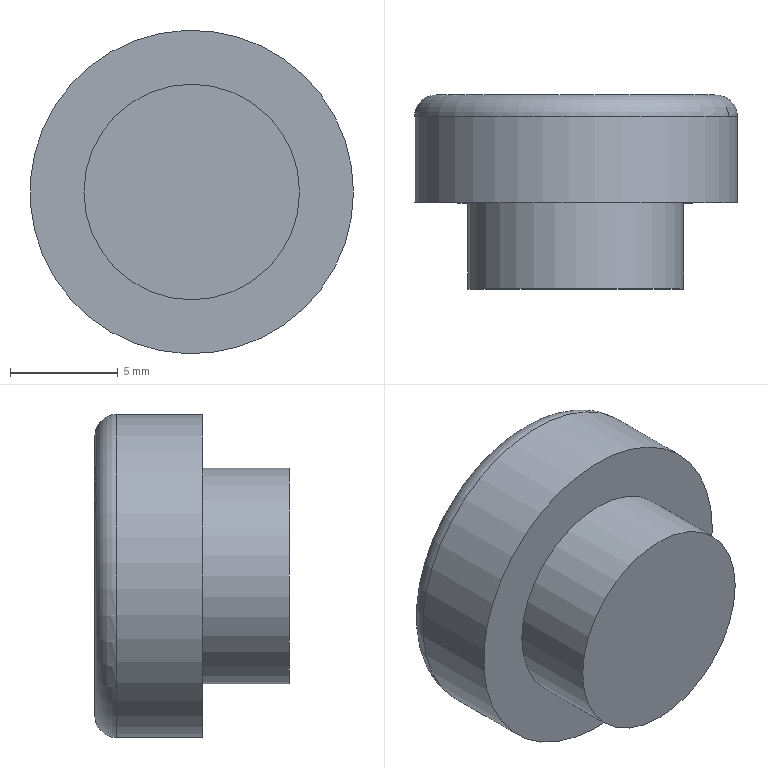Component | NX | BOLT | 1 solid | 6 faces | box 15 x 9 x 15 mm | volume 1188 mm3 | plane 3 | cylinder 2 | torus 1 | commonest cylinder face diameters 15 x1 10 x1
STEP:
#1=CARTESIAN_POINT('',(0.,0.,0.));
#2=DIRECTION('',(0.,0.,1.));
#3=DIRECTION('',(1.,0.,0.));
#4=AXIS2_PLACEMENT_3D('',#1,#2,#3);
#5=CARTESIAN_POINT('',(289.193,16.,95.));
#6=VERTEX_POINT('',#5);
#7=CARTESIAN_POINT('',(281.693,16.,95.));
#8=DIRECTION('',(0.,-1.,0.));
#9=DIRECTION('',(1.,0.,0.));
#10=AXIS2_PLACEMENT_3D('',#7,#8,#9);
#11=CIRCLE('',#10,7.5);
#12=CARTESIAN_POINT('',(281.693,17.,95.));
#13=DIRECTION('',(0.,-1.,0.));
#14=DIRECTION('',(-1.,0.,0.));
#15=AXIS2_PLACEMENT_3D('',#12,#13,#14);
#16=CYLINDRICAL_SURFACE('',#15,7.5);
#17=CARTESIAN_POINT('',(3.142,1.));
#18=DIRECTION('',(1.,0.));
#19=VECTOR('',#18,1.);
#20=LINE('',#17,#19);
#21=(GEOMETRIC_REPRESENTATION_CONTEXT(2)PARAMETRIC_REPRESENTATION_CONTEXT()REPRESENTATION_CONTEXT('',''));
#22=DEFINITIONAL_REPRESENTATION('',(#20),#21);
#23=PCURVE('',#16,#22);
#24=CARTESIAN_POINT('',(281.693,16.,95.));
#25=DIRECTION('',(0.,1.,0.));
#26=DIRECTION('',(1.,0.,0.));
#27=AXIS2_PLACEMENT_3D('',#24,#25,#26);
#28=TOROIDAL_SURFACE('',#27,6.5,1.);
#29=CARTESIAN_POINT('',(6.283,6.283));
#30=DIRECTION('',(-1.,0.));
#31=VECTOR('',#30,1.);
#32=LINE('',#29,#31);
#33=(GEOMETRIC_REPRESENTATION_CONTEXT(2)PARAMETRIC_REPRESENTATION_CONTEXT()REPRESENTATION_CONTEXT('',''));
#34=DEFINITIONAL_REPRESENTATION('',(#32),#33);
#35=PCURVE('',#28,#34);
#36=SURFACE_CURVE('',#11,(#23,#35),.PCURVE_S1.);
#37=EDGE_CURVE('',#6,#6,#36,.T.);
#38=ORIENTED_EDGE('',*,*,#37,.T.);
#39=CARTESIAN_POINT('',(289.193,12.,95.));
#40=VERTEX_POINT('',#39);
#41=CARTESIAN_POINT('',(289.193,16.,95.));
#42=CARTESIAN_POINT('',(289.193,12.,95.));
#43=B_SPLINE_CURVE_WITH_KNOTS('',1,(#41,#42),.UNSPECIFIED.,.F.,.F.,(2,2),(1.,5.),.PIECEWISE_BEZIER_KNOTS.);
#44=CARTESIAN_POINT('',(9.425,0.));
#45=DIRECTION('',(0.,1.));
#46=VECTOR('',#45,1.);
#47=LINE('',#44,#46);
#48=(GEOMETRIC_REPRESENTATION_CONTEXT(2)PARAMETRIC_REPRESENTATION_CONTEXT()REPRESENTATION_CONTEXT('',''));
#49=DEFINITIONAL_REPRESENTATION('',(#47),#48);
#50=PCURVE('',#16,#49);
#51=CARTESIAN_POINT('',(3.142,0.));
#52=DIRECTION('',(0.,1.));
#53=VECTOR('',#52,1.);
#54=LINE('',#51,#53);
#55=(GEOMETRIC_REPRESENTATION_CONTEXT(2)PARAMETRIC_REPRESENTATION_CONTEXT()REPRESENTATION_CONTEXT('',''));
#56=DEFINITIONAL_REPRESENTATION('',(#54),#55);
#57=PCURVE('',#16,#56);
#58=SEAM_CURVE('',#43,(#50,#57),.PCURVE_S1.);
#59=EDGE_CURVE('',#6,#40,#58,.T.);
#60=ORIENTED_EDGE('',*,*,#59,.T.);
#61=CARTESIAN_POINT('',(281.693,12.,95.));
#62=DIRECTION('',(0.,1.,0.));
#63=DIRECTION('',(1.,0.,0.));
#64=AXIS2_PLACEMENT_3D('',#61,#62,#63);
#65=CIRCLE('',#64,7.5);
#66=CARTESIAN_POINT('',(9.425,5.));
#67=DIRECTION('',(-1.,0.));
#68=VECTOR('',#67,1.);
#69=LINE('',#66,#68);
#70=(GEOMETRIC_REPRESENTATION_CONTEXT(2)PARAMETRIC_REPRESENTATION_CONTEXT()REPRESENTATION_CONTEXT('',''));
#71=DEFINITIONAL_REPRESENTATION('',(#69),#70);
#72=PCURVE('',#16,#71);
#73=CARTESIAN_POINT('',(281.693,12.,95.));
#74=DIRECTION('',(0.,1.,0.));
#75=DIRECTION('',(1.,0.,0.));
#76=AXIS2_PLACEMENT_3D('',#73,#74,#75);
#77=PLANE('',#76);
#78=CARTESIAN_POINT('',(0.,0.));
#79=DIRECTION('',(1.,0.));
#80=AXIS2_PLACEMENT_2D('',#78,#79);
#81=CIRCLE('',#80,7.5);
#82=(GEOMETRIC_REPRESENTATION_CONTEXT(2)PARAMETRIC_REPRESENTATION_CONTEXT()REPRESENTATION_CONTEXT('',''));
#83=DEFINITIONAL_REPRESENTATION('',(#81),#82);
#84=PCURVE('',#77,#83);
#85=SURFACE_CURVE('',#65,(#72,#84),.PCURVE_S1.);
#86=EDGE_CURVE('',#40,#40,#85,.T.);
#87=ORIENTED_EDGE('',*,*,#86,.T.);
#88=ORIENTED_EDGE('',*,*,#59,.F.);
#89=EDGE_LOOP('',(#38,#60,#87,#88));
#90=FACE_BOUND('',#89,.T.);
#91=ADVANCED_FACE('',(#90),#16,.T.);
#92=CARTESIAN_POINT('',(288.193,17.,95.));
#93=VERTEX_POINT('',#92);
#94=CARTESIAN_POINT('',(281.693,17.,95.));
#95=DIRECTION('',(0.,1.,0.));
#96=DIRECTION('',(1.,0.,0.));
#97=AXIS2_PLACEMENT_3D('',#94,#95,#96);
#98=CIRCLE('',#97,6.5);
#99=CARTESIAN_POINT('',(281.693,17.,95.));
#100=DIRECTION('',(0.,1.,0.));
#101=DIRECTION('',(1.,0.,0.));
#102=AXIS2_PLACEMENT_3D('',#99,#100,#101);
#103=PLANE('',#102);
#104=CARTESIAN_POINT('',(0.,0.));
#105=DIRECTION('',(1.,0.));
#106=AXIS2_PLACEMENT_2D('',#104,#105);
#107=CIRCLE('',#106,6.5);
#108=(GEOMETRIC_REPRESENTATION_CONTEXT(2)PARAMETRIC_REPRESENTATION_CONTEXT()REPRESENTATION_CONTEXT('',''));
#109=DEFINITIONAL_REPRESENTATION('',(#107),#108);
#110=PCURVE('',#103,#109);
#111=CARTESIAN_POINT('',(0.,7.854));
#112=DIRECTION('',(1.,0.));
#113=VECTOR('',#112,1.);
#114=LINE('',#111,#113);
#115=(GEOMETRIC_REPRESENTATION_CONTEXT(2)PARAMETRIC_REPRESENTATION_CONTEXT()REPRESENTATION_CONTEXT('',''));
#116=DEFINITIONAL_REPRESENTATION('',(#114),#115);
#117=PCURVE('',#28,#116);
#118=SURFACE_CURVE('',#98,(#110,#117),.PCURVE_S1.);
#119=EDGE_CURVE('',#93,#93,#118,.T.);
#120=ORIENTED_EDGE('',*,*,#119,.T.);
#121=EDGE_LOOP('',(#120));
#122=FACE_BOUND('',#121,.T.);
#123=ADVANCED_FACE('',(#122),#103,.T.);
#124=CARTESIAN_POINT('',(286.693,12.,95.));
#125=VERTEX_POINT('',#124);
#126=CARTESIAN_POINT('',(281.693,12.,95.));
#127=DIRECTION('',(0.,-1.,0.));
#128=DIRECTION('',(1.,0.,0.));
#129=AXIS2_PLACEMENT_3D('',#126,#127,#128);
#130=CIRCLE('',#129,5.);
#131=CARTESIAN_POINT('',(5.,0.));
#132=CARTESIAN_POINT('',(5.,-8.66));
#133=CARTESIAN_POINT('',(-2.5,-4.33));
#134=CARTESIAN_POINT('',(-10.,-0.));
#135=CARTESIAN_POINT('',(-2.5,4.33));
#136=CARTESIAN_POINT('',(5.,8.66));
#137=CARTESIAN_POINT('',(5.,0.));
#138=(BOUNDED_CURVE()B_SPLINE_CURVE(2,(#131,#132,#133,#134,#135,#136,#137),.UNSPECIFIED.,.T.,.F.)B_SPLINE_CURVE_WITH_KNOTS((1,2,2,2,2,1),(-2.094,0.,2.094,4.189,6.283,8.378),.UNSPECIFIED.)CURVE()GEOMETRIC_REPRESENTATION_ITEM()RATIONAL_B_SPLINE_CURVE((1.,0.5,1.,0.5,1.,0.5,1.))REPRESENTATION_ITEM(''));
#139=(GEOMETRIC_REPRESENTATION_CONTEXT(2)PARAMETRIC_REPRESENTATION_CONTEXT()REPRESENTATION_CONTEXT('',''));
#140=DEFINITIONAL_REPRESENTATION('',(#138),#139);
#141=PCURVE('',#77,#140);
#142=CARTESIAN_POINT('',(281.693,8.,95.));
#143=DIRECTION('',(0.,1.,0.));
#144=DIRECTION('',(1.,0.,0.));
#145=AXIS2_PLACEMENT_3D('',#142,#143,#144);
#146=CYLINDRICAL_SURFACE('',#145,5.);
#147=CARTESIAN_POINT('',(6.283,4.));
#148=DIRECTION('',(-1.,0.));
#149=VECTOR('',#148,1.);
#150=LINE('',#147,#149);
#151=(GEOMETRIC_REPRESENTATION_CONTEXT(2)PARAMETRIC_REPRESENTATION_CONTEXT()REPRESENTATION_CONTEXT('',''));
#152=DEFINITIONAL_REPRESENTATION('',(#150),#151);
#153=PCURVE('',#146,#152);
#154=SURFACE_CURVE('',#130,(#141,#153),.PCURVE_S1.);
#155=EDGE_CURVE('',#125,#125,#154,.T.);
#156=ORIENTED_EDGE('',*,*,#155,.F.);
#157=EDGE_LOOP('',(#156));
#158=FACE_BOUND('',#157,.T.);
#159=ORIENTED_EDGE('',*,*,#86,.F.);
#160=EDGE_LOOP('',(#159));
#161=FACE_BOUND('',#160,.T.);
#162=ADVANCED_FACE('',(#158,#161),#77,.F.);
#163=ORIENTED_EDGE('',*,*,#37,.F.);
#164=CARTESIAN_POINT('',(289.193,16.,95.));
#165=CARTESIAN_POINT('',(289.193,16.267,95.));
#166=CARTESIAN_POINT('',(289.108,16.528,95.));
#167=CARTESIAN_POINT('',(288.945,16.752,95.));
#168=CARTESIAN_POINT('',(288.72,16.915,95.));
#169=CARTESIAN_POINT('',(288.46,17.,95.));
#170=CARTESIAN_POINT('',(288.193,17.,95.));
#171=(BOUNDED_CURVE()B_SPLINE_CURVE(6,(#164,#165,#166,#167,#168,#169,#170),.UNSPECIFIED.,.F.,.F.)B_SPLINE_CURVE_WITH_KNOTS((7,7),(0.,1.571),.PIECEWISE_BEZIER_KNOTS.)CURVE()GEOMETRIC_REPRESENTATION_ITEM()RATIONAL_B_SPLINE_CURVE((1.031,1.01,0.9979,0.994,0.9979,1.01,1.031))REPRESENTATION_ITEM(''));
#172=CARTESIAN_POINT('',(6.283,6.283));
#173=DIRECTION('',(0.,1.));
#174=VECTOR('',#173,1.);
#175=LINE('',#172,#174);
#176=(GEOMETRIC_REPRESENTATION_CONTEXT(2)PARAMETRIC_REPRESENTATION_CONTEXT()REPRESENTATION_CONTEXT('',''));
#177=DEFINITIONAL_REPRESENTATION('',(#175),#176);
#178=PCURVE('',#28,#177);
#179=CARTESIAN_POINT('',(0.,6.283));
#180=DIRECTION('',(0.,1.));
#181=VECTOR('',#180,1.);
#182=LINE('',#179,#181);
#183=(GEOMETRIC_REPRESENTATION_CONTEXT(2)PARAMETRIC_REPRESENTATION_CONTEXT()REPRESENTATION_CONTEXT('',''));
#184=DEFINITIONAL_REPRESENTATION('',(#182),#183);
#185=PCURVE('',#28,#184);
#186=SEAM_CURVE('',#171,(#178,#185),.PCURVE_S1.);
#187=EDGE_CURVE('',#6,#93,#186,.T.);
#188=ORIENTED_EDGE('',*,*,#187,.T.);
#189=ORIENTED_EDGE('',*,*,#119,.F.);
#190=ORIENTED_EDGE('',*,*,#187,.F.);
#191=EDGE_LOOP('',(#163,#188,#189,#190));
#192=FACE_BOUND('',#191,.T.);
#193=ADVANCED_FACE('',(#192),#28,.T.);
#194=CARTESIAN_POINT('',(286.693,8.,95.));
#195=VERTEX_POINT('',#194);
#196=CARTESIAN_POINT('',(281.693,8.,95.));
#197=DIRECTION('',(0.,-1.,0.));
#198=DIRECTION('',(1.,0.,0.));
#199=AXIS2_PLACEMENT_3D('',#196,#197,#198);
#200=CIRCLE('',#199,5.);
#201=CARTESIAN_POINT('',(6.283,0.));
#202=DIRECTION('',(-1.,0.));
#203=VECTOR('',#202,1.);
#204=LINE('',#201,#203);
#205=(GEOMETRIC_REPRESENTATION_CONTEXT(2)PARAMETRIC_REPRESENTATION_CONTEXT()REPRESENTATION_CONTEXT('',''));
#206=DEFINITIONAL_REPRESENTATION('',(#204),#205);
#207=PCURVE('',#146,#206);
#208=CARTESIAN_POINT('',(281.693,8.,95.));
#209=DIRECTION('',(0.,-1.,0.));
#210=DIRECTION('',(-1.,0.,0.));
#211=AXIS2_PLACEMENT_3D('',#208,#209,#210);
#212=PLANE('',#211);
#213=CARTESIAN_POINT('',(0.,0.));
#214=DIRECTION('',(-1.,0.));
#215=AXIS2_PLACEMENT_2D('',#213,#214);
#216=CIRCLE('',#215,5.);
#217=(GEOMETRIC_REPRESENTATION_CONTEXT(2)PARAMETRIC_REPRESENTATION_CONTEXT()REPRESENTATION_CONTEXT('',''));
#218=DEFINITIONAL_REPRESENTATION('',(#216),#217);
#219=PCURVE('',#212,#218);
#220=SURFACE_CURVE('',#200,(#207,#219),.PCURVE_S1.);
#221=EDGE_CURVE('',#195,#195,#220,.T.);
#222=ORIENTED_EDGE('',*,*,#221,.F.);
#223=CARTESIAN_POINT('',(286.693,8.,95.));
#224=CARTESIAN_POINT('',(286.693,12.,95.));
#225=B_SPLINE_CURVE_WITH_KNOTS('',1,(#223,#224),.UNSPECIFIED.,.F.,.F.,(2,2),(0.,4.),.PIECEWISE_BEZIER_KNOTS.);
#226=CARTESIAN_POINT('',(6.283,0.));
#227=DIRECTION('',(0.,1.));
#228=VECTOR('',#227,1.);
#229=LINE('',#226,#228);
#230=(GEOMETRIC_REPRESENTATION_CONTEXT(2)PARAMETRIC_REPRESENTATION_CONTEXT()REPRESENTATION_CONTEXT('',''));
#231=DEFINITIONAL_REPRESENTATION('',(#229),#230);
#232=PCURVE('',#146,#231);
#233=CARTESIAN_POINT('',(0.,0.));
#234=DIRECTION('',(0.,1.));
#235=VECTOR('',#234,1.);
#236=LINE('',#233,#235);
#237=(GEOMETRIC_REPRESENTATION_CONTEXT(2)PARAMETRIC_REPRESENTATION_CONTEXT()REPRESENTATION_CONTEXT('',''));
#238=DEFINITIONAL_REPRESENTATION('',(#236),#237);
#239=PCURVE('',#146,#238);
#240=SEAM_CURVE('',#225,(#232,#239),.PCURVE_S1.);
#241=EDGE_CURVE('',#195,#125,#240,.T.);
#242=ORIENTED_EDGE('',*,*,#241,.T.);
#243=ORIENTED_EDGE('',*,*,#155,.T.);
#244=ORIENTED_EDGE('',*,*,#241,.F.);
#245=EDGE_LOOP('',(#222,#242,#243,#244));
#246=FACE_BOUND('',#245,.T.);
#247=ADVANCED_FACE('',(#246),#146,.T.);
#248=ORIENTED_EDGE('',*,*,#221,.T.);
#249=EDGE_LOOP('',(#248));
#250=FACE_BOUND('',#249,.T.);
#251=ADVANCED_FACE('',(#250),#212,.T.);
#252=CLOSED_SHELL('',(#91,#123,#162,#193,#247,#251));
#253=MANIFOLD_SOLID_BREP('',#252);
#254=(LENGTH_UNIT()NAMED_UNIT(*)SI_UNIT(.MILLI.,.METRE.));
#255=UNCERTAINTY_MEASURE_WITH_UNIT(LENGTH_MEASURE(0.00001),#254,'','');
#256=(NAMED_UNIT(*)PLANE_ANGLE_UNIT()SI_UNIT($,.RADIAN.));
#257=(NAMED_UNIT(*)SI_UNIT($,.STERADIAN.)SOLID_ANGLE_UNIT());
#258=(GEOMETRIC_REPRESENTATION_CONTEXT(3)GLOBAL_UNCERTAINTY_ASSIGNED_CONTEXT((#255))GLOBAL_UNIT_ASSIGNED_CONTEXT((#254,#256,#257))REPRESENTATION_CONTEXT('',''));
#259=ADVANCED_BREP_SHAPE_REPRESENTATION('',(#4,#253),#258);